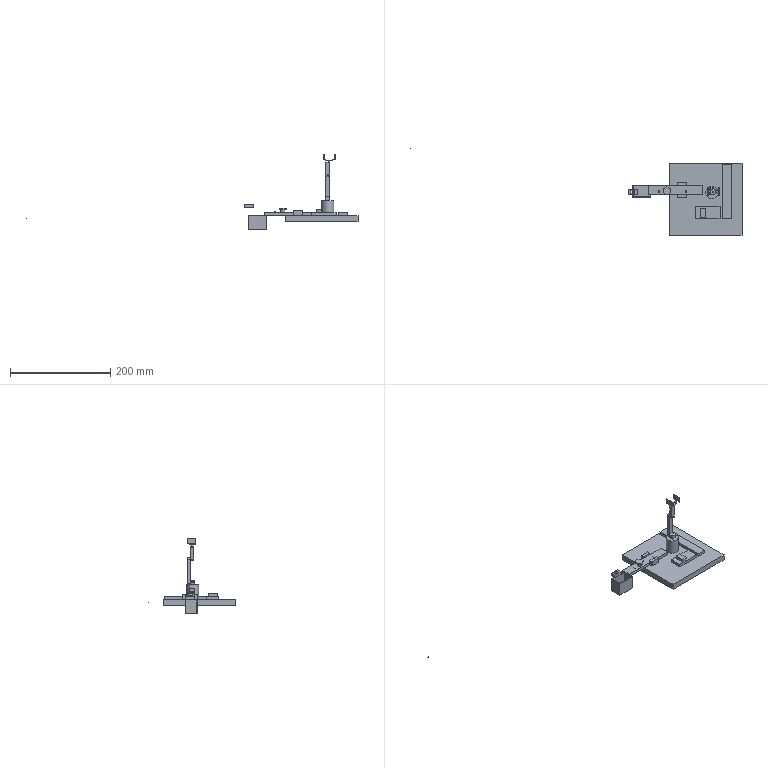Assembly | NX | mm | 19 component files | 19 solids | 149 faces | box 663.09 x 173.2 x 151.67 mm | volume 306514 mm3 | plane 132 | cylinder 17 | commonest cylinder face diameters 5 x8 2 x3 8.1 x1 8 x1 24 x1 2.5 x1 3 x1 12 x1
Bill of materials:
unnamed part 1 | 1 |  | Solid right circular cylinder with a smaller square-section boss centered on one flat end; the boss has a small round cross hole running through it from side to side.
unnamed part 2 | 1 |  | Thick, elongated flat bar with a rounded-rectangle profile and one small round through hole near one end.
unnamed part 3 | 1 |  | Very thin circular disc with a short solid cylindrical boss centered on one face, giving a flanged-pin or thin-headed shape.
unnamed part 4 | 1 |  | Rectangular block with one large round through hole running through its thickness, roughly centered on the largest face.
unnamed part 5 | 3 |  | Plain solid rectangular block with no visible holes or features.
unnamed part 6 | 2 |  | Thin, plain rectangular plate or strip with no visible holes or features.
unnamed part 7 | 1 |  | Plain flat rectangular slab of moderate thickness with no visible features.
unnamed part 8 | 2 |  | Thin rectangular plate that, according to the orthographic views, has a smaller rectangular block or tab sticking out from one face near one edge.
unnamed part 9 | 1 |  | Thin, plain square (or nearly square) plate with no visible holes or features.
unnamed part 10 | 1 |  | Plain solid rectangular block, thick plate-like, with two face dimensions that are nearly equal and a smaller thickness.
unnamed part 11 | 1 |  | Thin-walled, open-top rectangular box or tray: four vertical walls around a rectangular opening.
unnamed part 12 | 1 |  | Hexagonal prism head with a short plain cylindrical shank centered underneath, like a hex-headed bolt or plug.
unnamed part 13 | 1 |  | Elongated, thick bar-like block. Its main outline is a long rectangle with rounded corners. There is one small round hole near each end, and the edges are rounded.
unnamed part 14 | 2 |  | Plain, solid rectangular flat bar (a rectangular block) with no visible holes, cutouts or other features.
Mates:
1. touch align | transfer_surface 1 edge | transfer_surface_32 2 edge
2. fix | robot_arm_base 1 component
3. fix | large_base_plate 1 component
4. fix | transfer_surface 1 component
5. fix | workpiece_raw_1 3 component
6. touch align | robot_arm_long_arm 1 edge | robot_arm_base 1 line
7. align lock | robot_arm_long_arm 1 edge | robot_arm_base 1 edge
8. concentric | robot_arm_short_arm 1 edge | robot_arm_long_arm 1 edge
9. touch align | robot_arm_flange 1 edge | robot_arm_short_arm 1 edge
10. fix | robot_arm_flange 1 component
11. fix | gripper_21 2 component
12. align lock | workpiece_raw_1 1 edge | transfer_surface_32 1 edge
13. align lock | workpiece_raw_1 2 edge | transfer_surface_32 1 edge